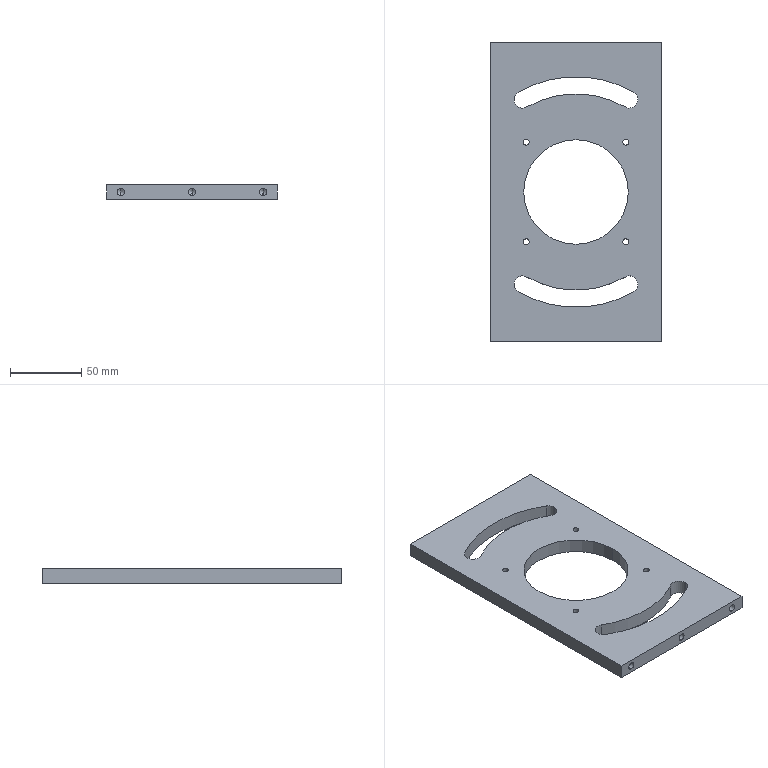Component | SolidWorks | 75-02-12StirringMountingPlate-1 | 1 solid | 50 faces | box 120 x 210 x 10 mm | volume 186079 mm3 | cylinder 32 | cone 12 | plane 6 | commonest cylinder face diameters 5 x12 4.2 x8 12 x6 73.5 x2 138 x2 162 x2 | material A3 Steel
build123d program:
from build123d import *

# Parameters (mm, degrees)
SKETCH1_W                  = 120
SKETCH1_H                  = 210
BOSS_EXTRUDE1_DEPTH        = 5
M6_TAPPED_HOLE1_AT_2_COUNT = 2
M6_TAPPED_HOLE1_AT_2_PITCH = 100
M6_TAPPED_HOLE1_AT_3_COUNT = 2
M6_TAPPED_HOLE1_AT_3_PITCH = 50
SKETCH5_R                  = 36.75
CUT_EXTRUDE1_DEPTH         = 122.347
M5_TAPPED_HOLE1_D          = 4.2
CUT_EXTRUDE2_DEPTH         = 122.347


with BuildPart() as part:
    # Sketch1 → Boss-Extrude1 (new, symmetric)
    with BuildSketch(Plane.XY):
        Rectangle(SKETCH1_W, SKETCH1_H)
    extrude(amount=BOSS_EXTRUDE1_DEPTH, both=True)

    # Sketch4 → M6 Tapped Hole1 (revolve, cut)
    with BuildSketch(Plane(origin=(-50, 105, 0), x_dir=(0, 0, 1), z_dir=(1, 0, 0))):
        Polygon((0, 0), (0, 16.502), (2.5, 15), (2.5, 0), align=None)
    m6_tapped_hole1 = revolve(axis=Axis((-50, 111.35, 0), (0, -1, 0)), mode=Mode.SUBTRACT)

    # M6 Tapped Hole1 at 2: M6 Tapped Hole1 ×2
    with Locations(*[(i * M6_TAPPED_HOLE1_AT_2_PITCH, 0, 0) for i in range(1, M6_TAPPED_HOLE1_AT_2_COUNT)]):
        add(m6_tapped_hole1, mode=Mode.SUBTRACT)

    # M6 Tapped Hole1 at 3: M6 Tapped Hole1 ×2
    with Locations(*[(i * M6_TAPPED_HOLE1_AT_3_PITCH, 0, 0) for i in range(1, M6_TAPPED_HOLE1_AT_3_COUNT)]):
        add(m6_tapped_hole1, mode=Mode.SUBTRACT)

    # Mirror1: M6 Tapped Hole1 across plane
    add(m6_tapped_hole1.mirror(Plane.ZX), mode=Mode.SUBTRACT)

    # Mirror1 copy 1 sketch → Mirror1 copy 1 (revolve, cut)
    with BuildSketch(Plane(origin=(50, -105, 0), x_dir=(0, 0, 1), z_dir=(1, 0, 0))):
        Polygon((0, 0), (0, -16.502), (2.5, -15), (2.5, 0), align=None)
    revolve(axis=Axis((50, -111.35, 0), (0, -1, 0)), mode=Mode.SUBTRACT)

    # Mirror1 copy 2 sketch → Mirror1 copy 2 (revolve, cut)
    with BuildSketch(Plane(origin=(0, -105, 0), x_dir=(0, 0, 1), z_dir=(1, 0, 0))):
        Polygon((0, 0), (0, -16.502), (2.5, -15), (2.5, 0), align=None)
    revolve(axis=Axis((0, -111.35, 0), (0, -1, 0)), mode=Mode.SUBTRACT)

    # Sketch5 → Cut-Extrude1 (cut, through all)
    with BuildSketch(Plane.XY.offset(5)):
        Circle(SKETCH5_R)
    extrude(amount=-CUT_EXTRUDE1_DEPTH, mode=Mode.SUBTRACT)

    # M5 Tapped Hole1 (through all)
    with Locations(Plane(origin=(-35, 35, 5), x_dir=(1, 0, 0), z_dir=(0, 0, 1))):
        with Locations((0, 0), (70, 0), (70, -70), (0, -70)):
            Hole(M5_TAPPED_HOLE1_D / 2)

    # Sketch9 → Cut-Extrude2 (cut, through all)
    with BuildSketch(Plane.XY.offset(5)):
        with BuildLine():
            ThreePointArc((40.5, 70.148), (0, 81), (-40.5, 70.148))
            ThreePointArc((-40.5, 70.148), (-42.696, 61.952), (-34.5, 59.756))
            ThreePointArc((-34.5, 59.756), (0, 69), (34.5, 59.756))
            ThreePointArc((34.5, 59.756), (42.696, 61.952), (40.5, 70.148))
        make_face()
    cut_extrude2 = extrude(amount=-CUT_EXTRUDE2_DEPTH, mode=Mode.SUBTRACT)

    # Mirror2: Cut-Extrude2 across plane
    add(cut_extrude2.mirror(Plane.ZX), mode=Mode.SUBTRACT)


solid = part.part

# Placed as in the assembly
solid = solid.moved(Location((-17.8, 11.867, 107.75), (0, 0, 0)))